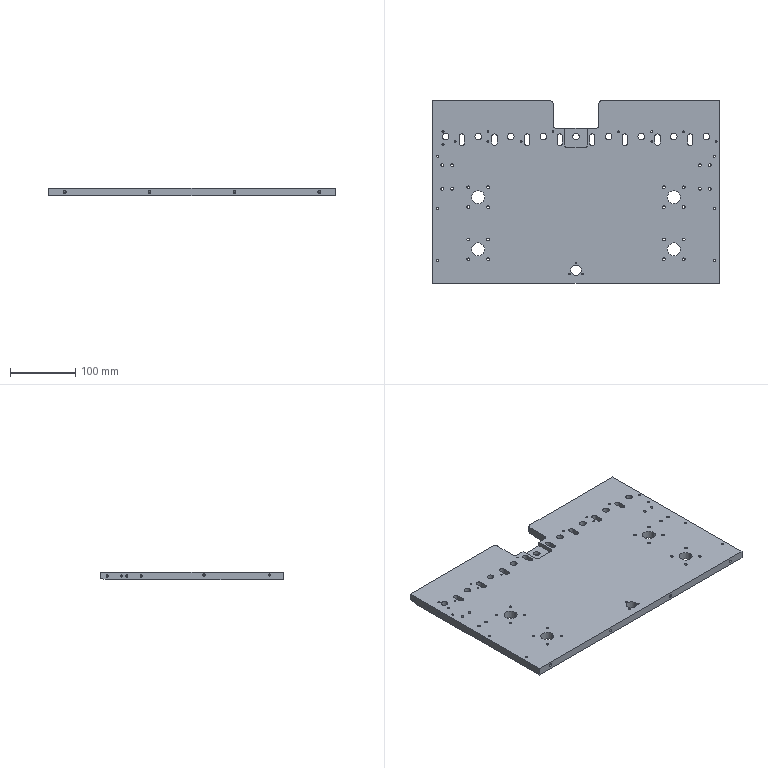Component | SolidWorks | 002MaterialPickingModuleA-1_J-002-1 | 1 solid | 236 faces | box 440 x 280 x 12 mm | volume 1385112 mm3 | cylinder 172 | cone 32 | plane 32 | commonest cylinder face diameters 4.2 x56 3.3 x40 2.5 x22 10 x22 8 x16 20 x8 3 x4 16 x2 | material 45
build123d program:
from build123d import *

# Parameters (mm, degrees)
SKETCH1_W                 = 440
SKETCH1_H                 = 280
BOSS_EXTRUDE1_DEPTH       = 12
SKETCH2_R                 = 10
CUT_EXTRUDE4_DEPTH        = 262.044
M5_TAPPED_HOLE1_D         = 4.2
SIZE_MM_DOWEL_PIN_HOLE1_D = 10
CUT_EXTRUDE5_DEPTH        = 262.044
LPATTERN1_COUNT           = 8
LPATTERN1_PITCH           = 50
SKETCH8_W                 = 70
SKETCH8_H                 = 85
CUT_EXTRUDE6_DEPTH        = 262.044
FILLET2_R                 = 5
SKETCH9_W                 = 34.2
SKETCH9_H                 = 30
CUT_EXTRUDE7_DEPTH        = 6.5
FILLET3_R                 = 3
M5_TAPPED_HOLE2_D         = 4.2
SKETCH12_R                = 8
CUT_EXTRUDE8_DEPTH        = 262.044
M3_TAPPED_HOLE1_D         = 2.5
CIRPATTERN1_COUNT         = 3
M4_TAPPED_HOLE2_D         = 3.3
M5_TAPPED_HOLE3_D         = 4.2
M5_TAPPED_HOLE3_DEPTH     = 12.4
M5_TAPPED_HOLE3_TIP       = 1.262
M4_TAPPED_HOLE3_D         = 3.3
M4_TAPPED_HOLE3_DEPTH     = 10.1
M4_TAPPED_HOLE3_TIP       = 0.9914
M4_TAPPED_HOLE4_D         = 3.3
M4_TAPPED_HOLE4_DEPTH     = 10.1
M4_TAPPED_HOLE4_TIP       = 0.9914
M4_TAPPED_HOLE5_D         = 3.3
M4_TAPPED_HOLE5_DEPTH     = 10.1
M4_TAPPED_HOLE5_TIP       = 0.9914
M3_TAPPED_HOLE2_D         = 2.5
SIZE_MM_DOWEL_PIN_HOLE2_D = 3
M4_TAPPED_HOLE6_D         = 3.3
M4_TAPPED_HOLE6_DEPTH     = 12.1
M4_TAPPED_HOLE6_TIP       = 0.9914
CHAMFER1_SIZE             = 15
CHAMFER1_SIZE2            = 2
FILLET4_R                 = 5
M4_TAPPED_HOLE7_D         = 3.3
M4_TAPPED_HOLE7_DEPTH     = 10.1
M4_TAPPED_HOLE7_TIP       = 0.9914
M4_TAPPED_HOLE8_D         = 3.3


with BuildPart() as part:
    # Sketch1 → Boss-Extrude1 (new body)
    with BuildSketch(Plane.XY):
        Rectangle(SKETCH1_W, SKETCH1_H)
    extrude(amount=BOSS_EXTRUDE1_DEPTH)

    # Sketch2 → Cut-Extrude4 (cut, through all)
    with BuildSketch(Plane.XY.offset(12)):
        with Locations((-150, -8)):
            Circle(SKETCH2_R)
        with Locations((150, -8)):
            Circle(SKETCH2_R)
        with Locations((-150, -88)):
            Circle(SKETCH2_R)
        with Locations((150, -88)):
            Circle(SKETCH2_R)
    extrude(amount=-CUT_EXTRUDE4_DEPTH, mode=Mode.SUBTRACT)

    # M5 Tapped Hole1 (through all)
    with Locations(Plane.XY.offset(12)):
        with Locations((-165.203, 7.203), (-165.203, -23.203), (-134.797, -23.203), (-134.797, 7.203), (-165.203, -72.797), (-134.797, -72.797), (-165.203, -103.203), (-134.797, -103.203), (134.797, -103.203), (165.203, -103.203), (134.797, -72.797), (165.203, -72.797), (134.797, -23.203), (165.203, -23.203), (134.797, 7.203), (165.203, 7.203)):
            Hole(M5_TAPPED_HOLE1_D / 2)

    # Size mm Dowel Pin Hole1 (through all)
    with Locations(Plane.XY.offset(12)):
        with Locations((0, 85), (-50, 85), (-100, 85), (-150, 85), (-200, 85), (50, 85), (100, 85), (150, 85), (200, 85)):
            Hole(SIZE_MM_DOWEL_PIN_HOLE1_D / 2)

    # Sketch7 → Cut-Extrude5 (cut, through all)
    with BuildSketch(Plane.XY.offset(12)):
        with BuildLine():
            Line((-171, 85), (-171, 75))
            ThreePointArc((-171, 75), (-175, 71), (-179, 75))
            Line((-179, 75), (-179, 85))
            ThreePointArc((-179, 85), (-175, 89), (-171, 85))
        make_face()
    cut_extrude5 = extrude(amount=-CUT_EXTRUDE5_DEPTH, mode=Mode.SUBTRACT)

    # LPattern1: Cut-Extrude5 ×8
    with Locations(*[(i * LPATTERN1_PITCH, 0, 0) for i in range(1, LPATTERN1_COUNT)]):
        add(cut_extrude5, mode=Mode.SUBTRACT)

    # Sketch8 → Cut-Extrude6 (cut, through all)
    with BuildSketch(Plane.XY.offset(12)):
        with Locations((0, 140)):
            Rectangle(SKETCH8_W, SKETCH8_H)
    extrude(amount=-CUT_EXTRUDE6_DEPTH, mode=Mode.SUBTRACT)

    # Fillet2
    fillet2_edges = [part.edges().sort_by_distance(p)[0] for p in [
        (-35, 97.5, 6),
        (35, 97.5, 6),
    ]]
    fillet(fillet2_edges, radius=FILLET2_R)

    # Sketch9 → Cut-Extrude7 (cut)
    with BuildSketch(Plane.XY.offset(12)):
        with Locations((0, 82.5)):
            Rectangle(SKETCH9_W, SKETCH9_H)
    extrude(amount=-CUT_EXTRUDE7_DEPTH, mode=Mode.SUBTRACT)

    # Fillet3
    fillet3_edges = [part.edges().sort_by_distance(p)[0] for p in [
        (-17.1, 67.5, 8.75),
        (17.1, 67.5, 8.75),
    ]]
    fillet(fillet3_edges, radius=FILLET3_R)

    # M5 Tapped Hole2 (through all)
    with Locations(Plane.XY.offset(12)):
        with Locations((190, 41), (205, 41), (190, 5), (205, 5)):
            m5_tapped_hole2 = Hole(M5_TAPPED_HOLE2_D / 2)

    # Mirror1: M5 Tapped Hole2 across plane
    add(m5_tapped_hole2.mirror(Plane(origin=(0, 0, 0), x_dir=(0, 0, 1), z_dir=(1, 0, 0))), mode=Mode.SUBTRACT)

    # Sketch12 → Cut-Extrude8 (cut, through all)
    with BuildSketch(Plane.XY.offset(12)):
        with Locations((0, -120)):
            Circle(SKETCH12_R)
    extrude(amount=-CUT_EXTRUDE8_DEPTH, mode=Mode.SUBTRACT)

    # M3 Tapped Hole1 (through all)
    with Locations(Plane.XY.offset(12)):
        with Locations((0, -109)):
            m3_tapped_hole1 = Hole(M3_TAPPED_HOLE1_D / 2)

    # CirPattern1: M3 Tapped Hole1 ×3 about axis
    cirpattern1_axis = Axis((0, -120, 0), (0, 0, 1))
    for i in range(1, CIRPATTERN1_COUNT):
        add(m3_tapped_hole1.rotate(cirpattern1_axis, i * 360 / CIRPATTERN1_COUNT), mode=Mode.SUBTRACT)

    # M4 Tapped Hole2 (through all)
    with Locations(Plane.XY.offset(12)):
        with Locations((-204, 73), (-204, 93)):
            Hole(M4_TAPPED_HOLE2_D / 2)

    # M5 Tapped Hole3
    with Locations(Plane(origin=(0, -140, 0), x_dir=(-1, 0, 0), z_dir=(0, -1, 0))):
        with Locations((65, -6), (-65, -6), (-195, -6), (195, -6)):
            Hole(M5_TAPPED_HOLE3_D / 2, depth=M5_TAPPED_HOLE3_DEPTH)
            with Locations((0, 0, -(M5_TAPPED_HOLE3_DEPTH + M5_TAPPED_HOLE3_TIP / 2))):  # 118° drill point
                Cone(0, M5_TAPPED_HOLE3_D / 2, M5_TAPPED_HOLE3_TIP, mode=Mode.SUBTRACT)

    # M4 Tapped Hole3
    with Locations(Plane(origin=(220, 0, 0), x_dir=(0, 0, -1), z_dir=(1, 0, 0))):
        with Locations((-7.5, -18.5), (-7.5, -118.5)):
            Hole(M4_TAPPED_HOLE3_D / 2, depth=M4_TAPPED_HOLE3_DEPTH)
            with Locations((0, 0, -(M4_TAPPED_HOLE3_DEPTH + M4_TAPPED_HOLE3_TIP / 2))):  # 118° drill point
                Cone(0, M4_TAPPED_HOLE3_D / 2, M4_TAPPED_HOLE3_TIP, mode=Mode.SUBTRACT)

    # M4 Tapped Hole4
    with Locations(Plane.ZY.offset(220)):
        with Locations((7.5, -18.5), (7.5, -118.5)):
            Hole(M4_TAPPED_HOLE4_D / 2, depth=M4_TAPPED_HOLE4_DEPTH)
            with Locations((0, 0, -(M4_TAPPED_HOLE4_DEPTH + M4_TAPPED_HOLE4_TIP / 2))):  # 118° drill point
                Cone(0, M4_TAPPED_HOLE4_D / 2, M4_TAPPED_HOLE4_TIP, mode=Mode.SUBTRACT)

    # M4 Tapped Hole5
    with Locations(Plane(origin=(0, 140, 0), x_dir=(1, 0, 0), z_dir=(0, 1, 0))):
        with Locations((-180, -7.5), (-60, -7.5), (60, -7.5), (180, -7.5)):
            Hole(M4_TAPPED_HOLE5_D / 2, depth=M4_TAPPED_HOLE5_DEPTH)
            with Locations((0, 0, -(M4_TAPPED_HOLE5_DEPTH + M4_TAPPED_HOLE5_TIP / 2))):  # 118° drill point
                Cone(0, M4_TAPPED_HOLE5_D / 2, M4_TAPPED_HOLE5_TIP, mode=Mode.SUBTRACT)

    # M3 Tapped Hole2 (through all)
    with Locations(Plane.XY.offset(12)):
        with Locations((-185, 77.5), (-135, 92.5), (-84.05, 77.5), (-35, 92.5), (115.95, 77.5), (165, 92.5), (215, 77.5), (65, 92.5)):
            Hole(M3_TAPPED_HOLE2_D / 2)

    # Size mm Dowel Pin Hole2 (through all)
    with Locations(Plane.XY.offset(12)):
        with Locations((115.95, 92.5), (-135, 77.5)):
            Hole(SIZE_MM_DOWEL_PIN_HOLE2_D / 2)

    # M4 Tapped Hole6
    with Locations(Plane.ZY.offset(220)):
        with Locations((6, 130), (6, 100)):
            Hole(M4_TAPPED_HOLE6_D / 2, depth=M4_TAPPED_HOLE6_DEPTH)
            with Locations((0, 0, -(M4_TAPPED_HOLE6_DEPTH + M4_TAPPED_HOLE6_TIP / 2))):  # 118° drill point
                Cone(0, M4_TAPPED_HOLE6_D / 2, M4_TAPPED_HOLE6_TIP, mode=Mode.SUBTRACT)

    # Chamfer1
    chamfer1_edges = [part.edges().sort_by_distance(p)[0] for p in [
        (-127.5, 140, 0),
        (127.5, 140, 0),
    ]]
    chamfer1_side = [part.faces().sort_by_distance(p)[0] for p in [
        (0.02595, -3.493, 0),
    ]]
    chamfer(chamfer1_edges, length=CHAMFER1_SIZE, length2=CHAMFER1_SIZE2, reference=chamfer1_side[0])

    # Fillet4
    fillet4_edges = [part.edges().sort_by_distance(p)[0] for p in [
        (-35, 140, 7),
        (35, 140, 7),
    ]]
    fillet(fillet4_edges, radius=FILLET4_R)

    # M4 Tapped Hole7
    with Locations(Plane.ZY.offset(220)):
        with Locations((6, 108), (6, 78)):
            Hole(M4_TAPPED_HOLE7_D / 2, depth=M4_TAPPED_HOLE7_DEPTH)
            with Locations((0, 0, -(M4_TAPPED_HOLE7_DEPTH + M4_TAPPED_HOLE7_TIP / 2))):  # 118° drill point
                Cone(0, M4_TAPPED_HOLE7_D / 2, M4_TAPPED_HOLE7_TIP, mode=Mode.SUBTRACT)

    # M4 Tapped Hole8 (through all)
    with Locations(Plane(origin=(0, 0, 0), x_dir=(-1, 0, 0), z_dir=(0, 0, -1))):
        with Locations((-212, -105), (-212, -25), (-212, 55)):
            m4_tapped_hole8 = Hole(M4_TAPPED_HOLE8_D / 2)

    # Mirror2: M4 Tapped Hole8 across plane
    add(m4_tapped_hole8.mirror(Plane(origin=(0, 0, 0), x_dir=(0, 0, 1), z_dir=(1, 0, 0))), mode=Mode.SUBTRACT)


solid = part.part

# Placed as in the assembly
solid = solid.moved(Location((220.325, 211.019, 416.231), (0, 0, 0)))